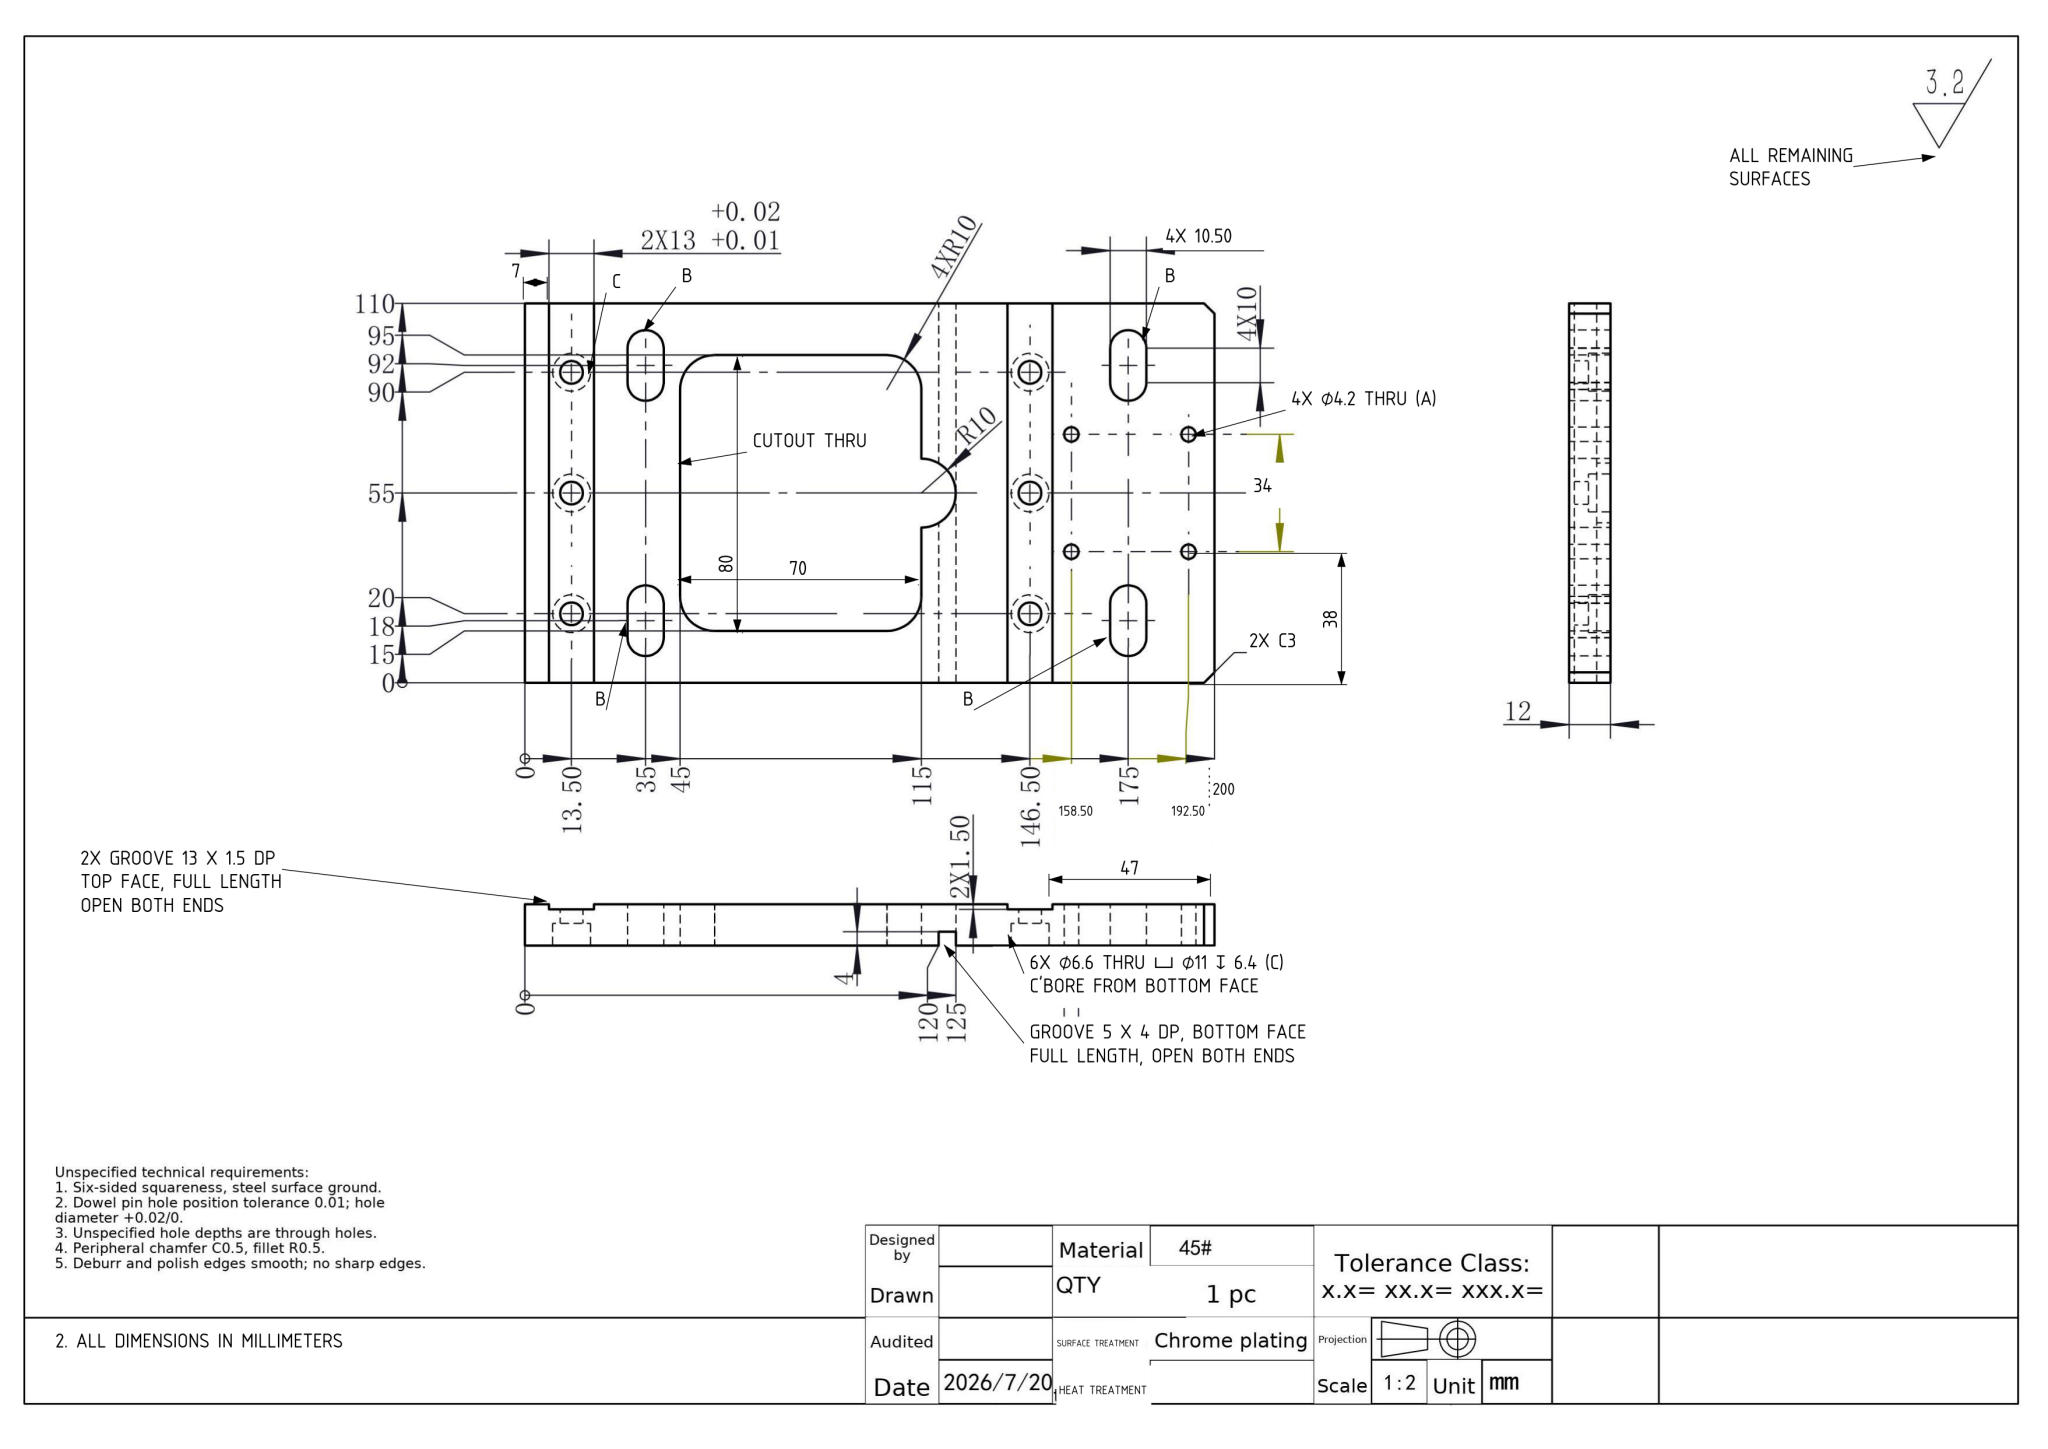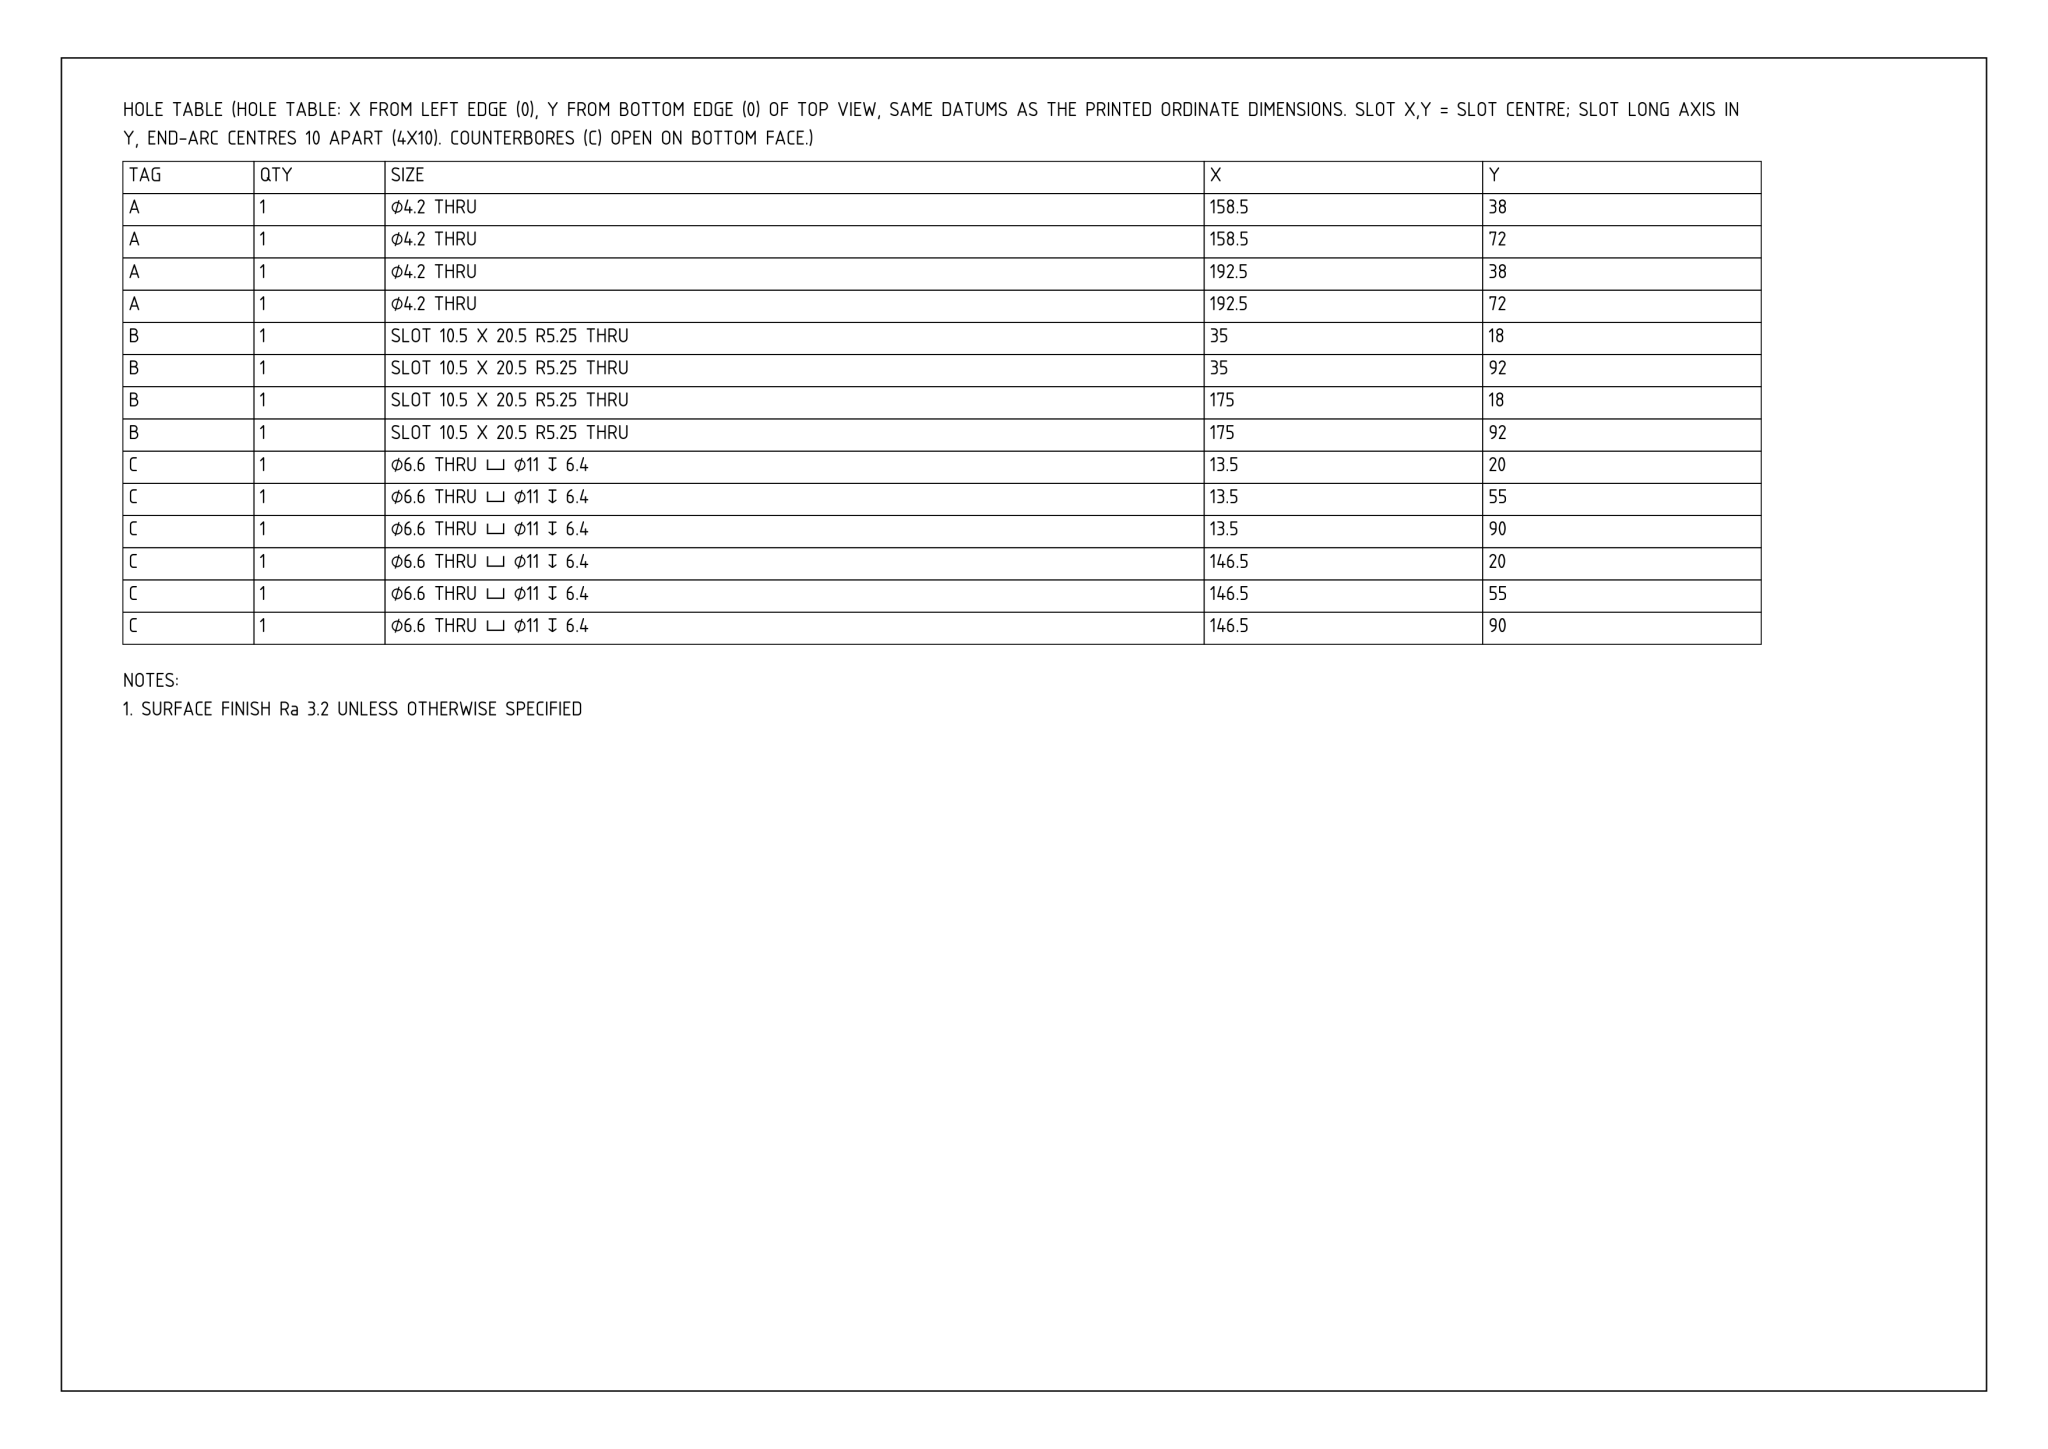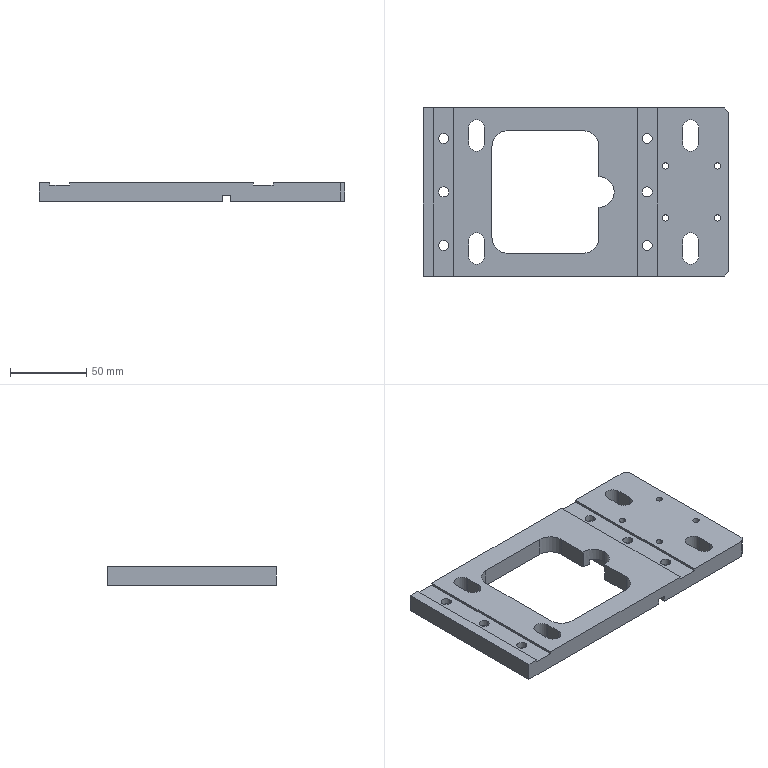Part | NX | mm | 1 solid | 87 faces | box 200 x 110 x 12 mm | volume 175241 mm3 | cylinder 46 | plane 41 | commonest cylinder face diameters 11 x12 6.6 x12 4.2 x8 10.5 x8 20 x6